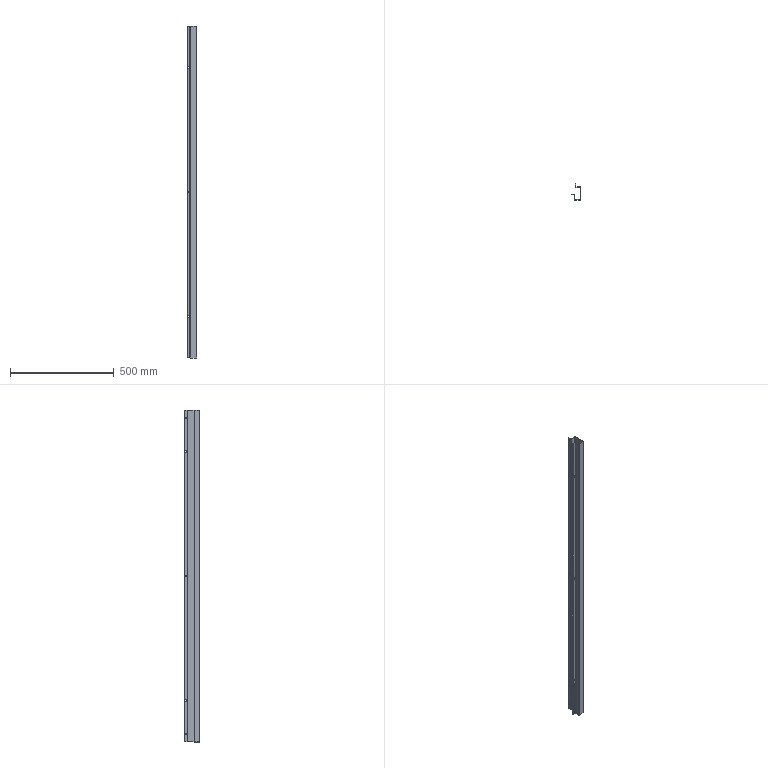Component | SolidWorks | Column-1 | 1 solid | 62 faces | volume 393880 mm3 | plane 36 | cylinder 26 | commonest cylinder face diameters 9.2 x12 5 x5 2 x5 5.4 x4